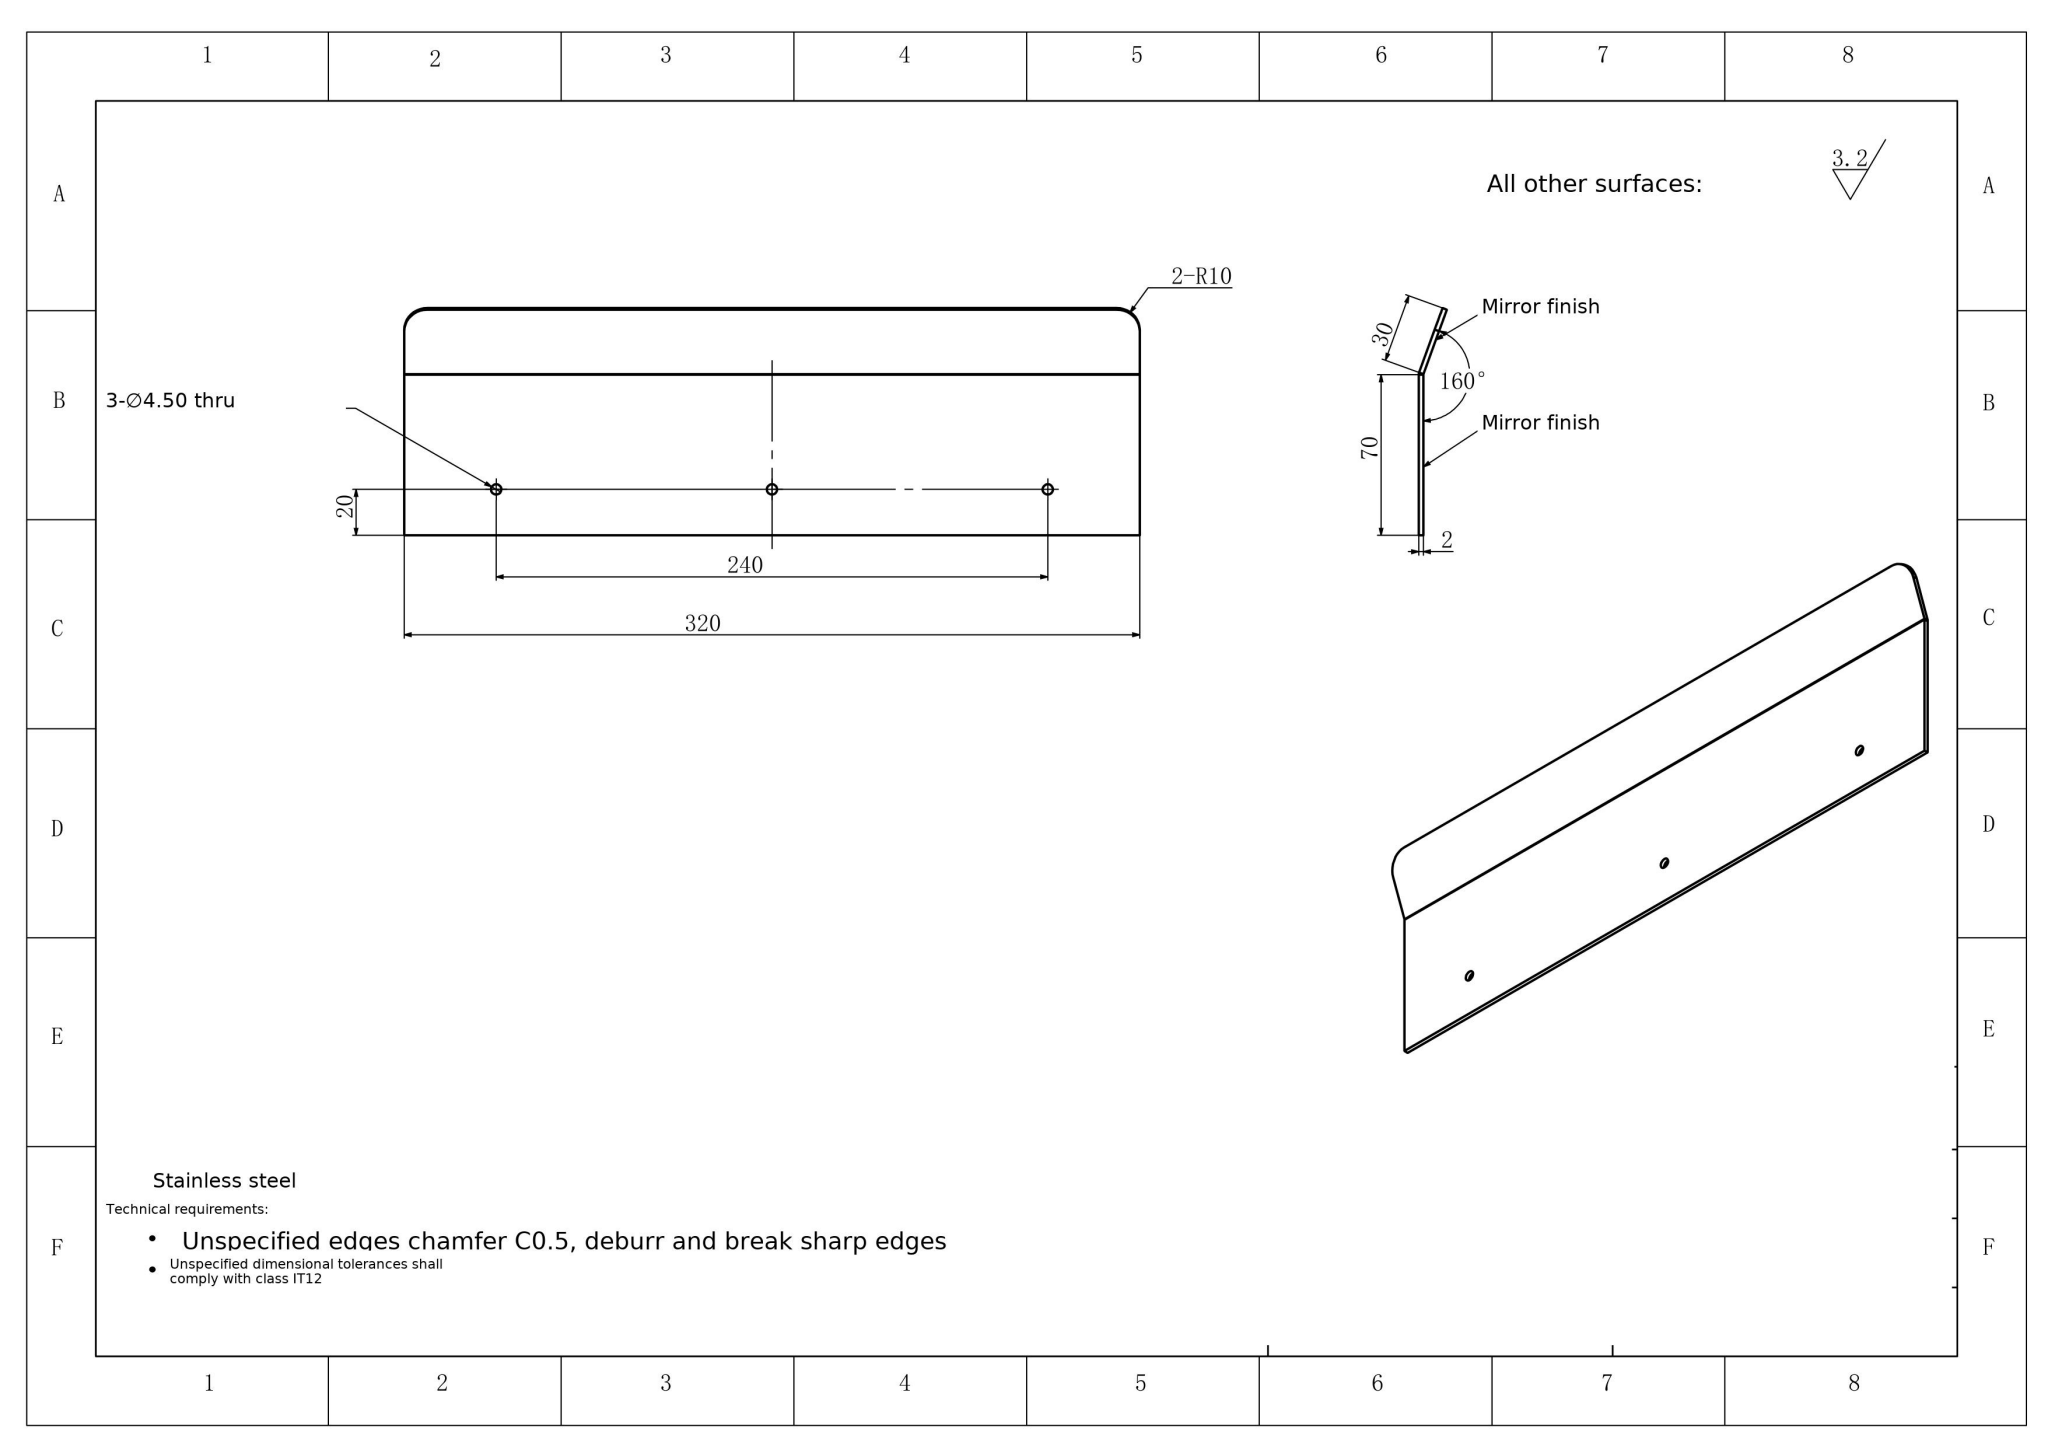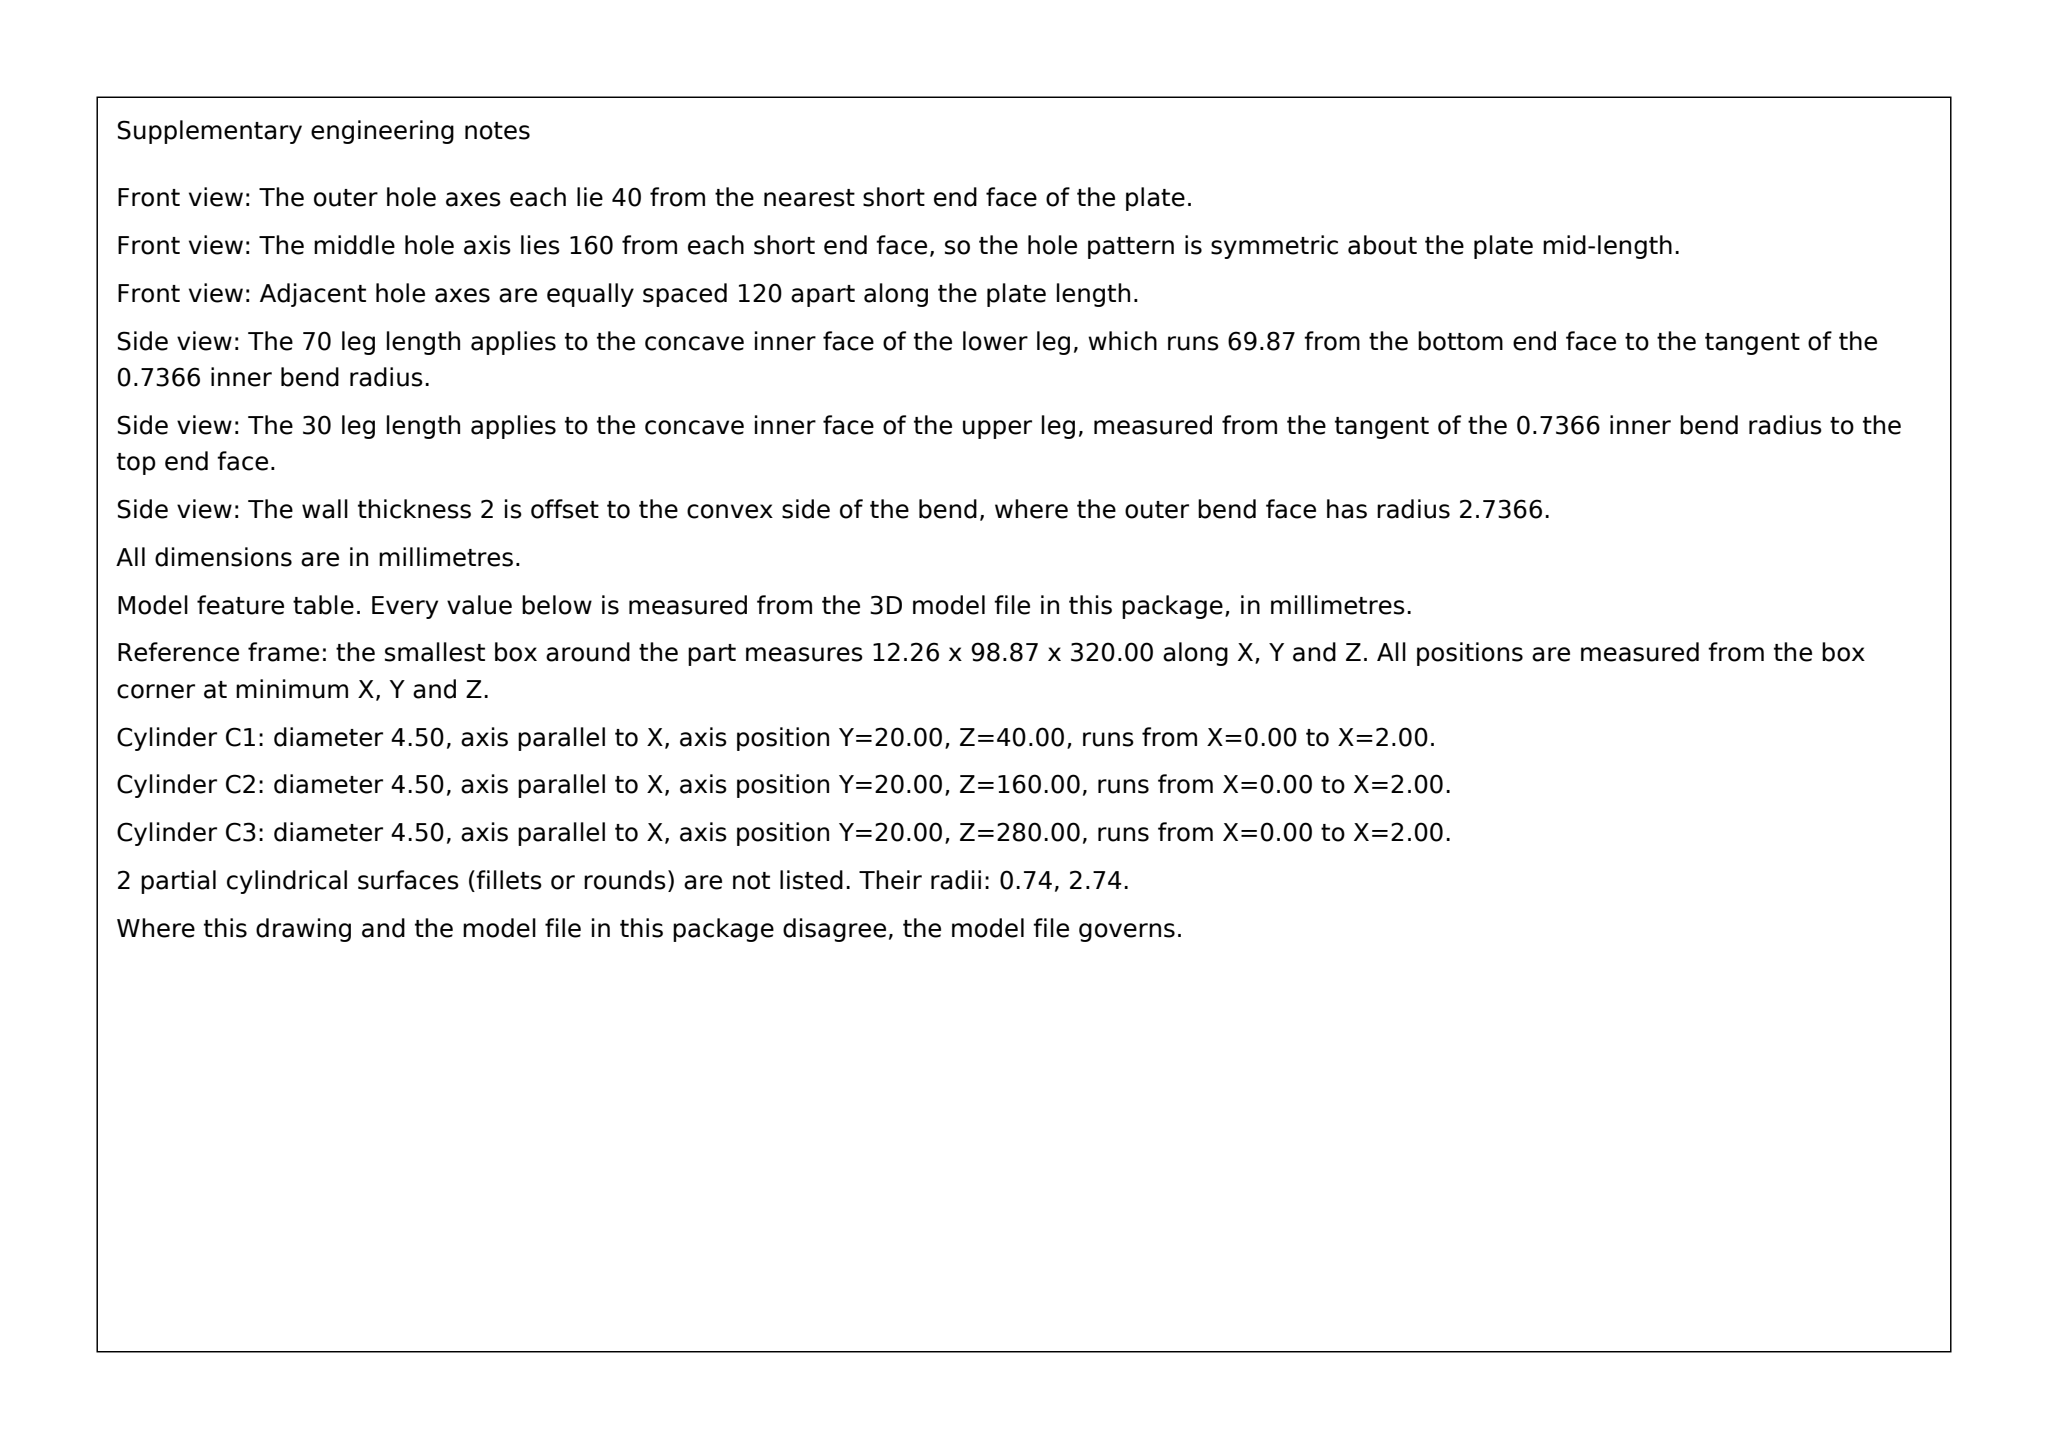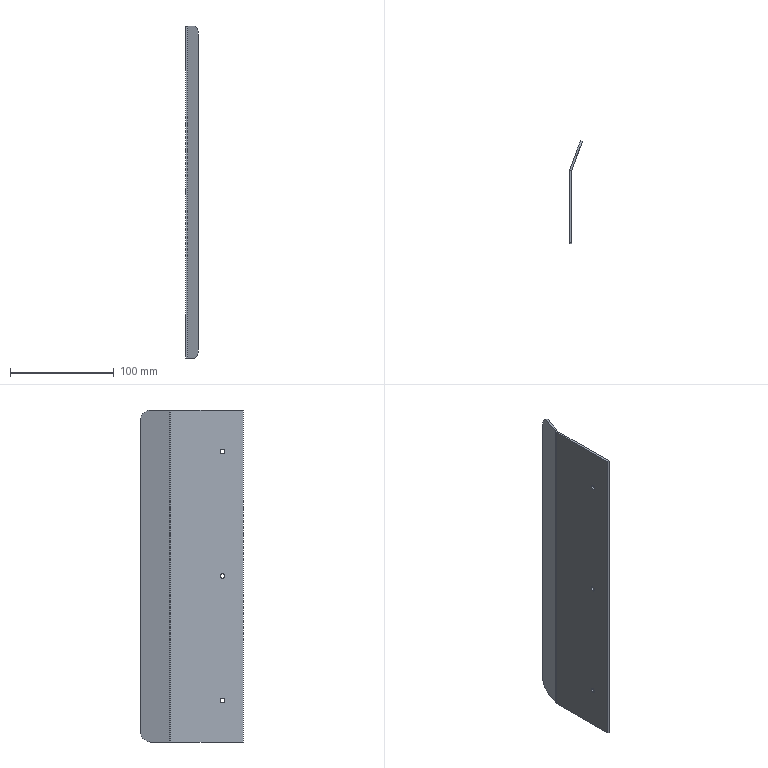Part | SolidWorks | mm | 1 solid | 22 faces | box 12.26 x 98.87 x 320 mm | volume 64040 mm3 | plane 12 | cylinder 10 | commonest cylinder face diameters 4.5 x6 20 x2 1.473 x1 5.473 x1
Drawing notes:
160° BEND: R0.74 INSIDE, R2.74 OUTSIDE | from the solid: cylinders dia 1.473 (r=0.7365) and 5.473 (r=2.736), axis z, len 320 at bend
ALL BENDS R0.74 INSIDE UNLESS NOTED; MATL THK 2 | from the solid: bend cyl dia 1.473 -> R0.74; planes x=0 and x=2.0 give 2 thk
STEP:
#1=CARTESIAN_POINT('',(-2.,-52.25,0.));
#2=VERTEX_POINT('',#1);
#3=CARTESIAN_POINT('',(-2.,-47.75,0.));
#4=VERTEX_POINT('',#3);
#5=CARTESIAN_POINT('',(-2.,-50.,0.));
#6=DIRECTION('',(1.,0.,0.));
#7=DIRECTION('',(-0.,1.,0.));
#8=AXIS2_PLACEMENT_3D('',#5,#6,#7);
#9=CIRCLE('',#8,2.25);
#10=EDGE_CURVE('',#2,#4,#9,.T.);
#11=ORIENTED_EDGE('',*,*,#10,.F.);
#12=CARTESIAN_POINT('',(0.,-52.25,0.));
#13=VERTEX_POINT('',#12);
#14=CARTESIAN_POINT('',(-10.,-52.25,0.));
#15=DIRECTION('',(1.,0.,0.));
#16=VECTOR('',#15,1000.);
#17=LINE('',#14,#16);
#18=EDGE_CURVE('',#2,#13,#17,.T.);
#19=ORIENTED_EDGE('',*,*,#18,.T.);
#20=CARTESIAN_POINT('',(0.,-47.75,0.));
#21=VERTEX_POINT('',#20);
#22=CARTESIAN_POINT('',(0.,-50.,0.));
#23=DIRECTION('',(1.,0.,0.));
#24=DIRECTION('',(-0.,1.,0.));
#25=AXIS2_PLACEMENT_3D('',#22,#23,#24);
#26=CIRCLE('',#25,2.25);
#27=EDGE_CURVE('',#13,#21,#26,.T.);
#28=ORIENTED_EDGE('',*,*,#27,.T.);
#29=CARTESIAN_POINT('',(-10.,-47.75,0.));
#30=DIRECTION('',(1.,0.,0.));
#31=VECTOR('',#30,1000.);
#32=LINE('',#29,#31);
#33=EDGE_CURVE('',#4,#21,#32,.T.);
#34=ORIENTED_EDGE('',*,*,#33,.F.);
#35=EDGE_LOOP('',(#11,#19,#28,#34));
#36=FACE_OUTER_BOUND('',#35,.T.);
#37=CARTESIAN_POINT('',(-10.,-50.,0.));
#38=DIRECTION('',(1.,0.,0.));
#39=DIRECTION('',(0.,1.,0.));
#40=AXIS2_PLACEMENT_3D('',#37,#38,#39);
#41=CYLINDRICAL_SURFACE('',#40,2.25);
#42=ADVANCED_FACE('',(#36),#41,.F.);
#43=CARTESIAN_POINT('',(-2.,-52.25,-120.));
#44=VERTEX_POINT('',#43);
#45=CARTESIAN_POINT('',(-2.,-47.75,-120.));
#46=VERTEX_POINT('',#45);
#47=CARTESIAN_POINT('',(-2.,-50.,-120.));
#48=DIRECTION('',(1.,0.,0.));
#49=DIRECTION('',(-0.,1.,0.));
#50=AXIS2_PLACEMENT_3D('',#47,#48,#49);
#51=CIRCLE('',#50,2.25);
#52=EDGE_CURVE('',#44,#46,#51,.T.);
#53=ORIENTED_EDGE('',*,*,#52,.F.);
#54=CARTESIAN_POINT('',(0.,-52.25,-120.));
#55=VERTEX_POINT('',#54);
#56=CARTESIAN_POINT('',(-10.,-52.25,-120.));
#57=DIRECTION('',(1.,0.,0.));
#58=VECTOR('',#57,1000.);
#59=LINE('',#56,#58);
#60=EDGE_CURVE('',#44,#55,#59,.T.);
#61=ORIENTED_EDGE('',*,*,#60,.T.);
#62=CARTESIAN_POINT('',(0.,-47.75,-120.));
#63=VERTEX_POINT('',#62);
#64=CARTESIAN_POINT('',(0.,-50.,-120.));
#65=DIRECTION('',(1.,0.,0.));
#66=DIRECTION('',(-0.,1.,0.));
#67=AXIS2_PLACEMENT_3D('',#64,#65,#66);
#68=CIRCLE('',#67,2.25);
#69=EDGE_CURVE('',#55,#63,#68,.T.);
#70=ORIENTED_EDGE('',*,*,#69,.T.);
#71=CARTESIAN_POINT('',(-10.,-47.75,-120.));
#72=DIRECTION('',(1.,0.,0.));
#73=VECTOR('',#72,1000.);
#74=LINE('',#71,#73);
#75=EDGE_CURVE('',#46,#63,#74,.T.);
#76=ORIENTED_EDGE('',*,*,#75,.F.);
#77=EDGE_LOOP('',(#53,#61,#70,#76));
#78=FACE_OUTER_BOUND('',#77,.T.);
#79=CARTESIAN_POINT('',(-10.,-50.,-120.));
#80=DIRECTION('',(1.,0.,0.));
#81=DIRECTION('',(0.,1.,0.));
#82=AXIS2_PLACEMENT_3D('',#79,#80,#81);
#83=CYLINDRICAL_SURFACE('',#82,2.25);
#84=ADVANCED_FACE('',(#78),#83,.F.);
#85=CARTESIAN_POINT('',(-2.,-52.25,120.));
#86=VERTEX_POINT('',#85);
#87=CARTESIAN_POINT('',(-2.,-47.75,120.));
#88=VERTEX_POINT('',#87);
#89=CARTESIAN_POINT('',(-2.,-50.,120.));
#90=DIRECTION('',(1.,0.,0.));
#91=DIRECTION('',(-0.,1.,0.));
#92=AXIS2_PLACEMENT_3D('',#89,#90,#91);
#93=CIRCLE('',#92,2.25);
#94=EDGE_CURVE('',#86,#88,#93,.T.);
#95=ORIENTED_EDGE('',*,*,#94,.F.);
#96=CARTESIAN_POINT('',(0.,-52.25,120.));
#97=VERTEX_POINT('',#96);
#98=CARTESIAN_POINT('',(-10.,-52.25,120.));
#99=DIRECTION('',(1.,0.,0.));
#100=VECTOR('',#99,1000.);
#101=LINE('',#98,#100);
#102=EDGE_CURVE('',#86,#97,#101,.T.);
#103=ORIENTED_EDGE('',*,*,#102,.T.);
#104=CARTESIAN_POINT('',(0.,-47.75,120.));
#105=VERTEX_POINT('',#104);
#106=CARTESIAN_POINT('',(0.,-50.,120.));
#107=DIRECTION('',(1.,0.,0.));
#108=DIRECTION('',(-0.,1.,0.));
#109=AXIS2_PLACEMENT_3D('',#106,#107,#108);
#110=CIRCLE('',#109,2.25);
#111=EDGE_CURVE('',#97,#105,#110,.T.);
#112=ORIENTED_EDGE('',*,*,#111,.T.);
#113=CARTESIAN_POINT('',(-10.,-47.75,120.));
#114=DIRECTION('',(1.,0.,0.));
#115=VECTOR('',#114,1000.);
#116=LINE('',#113,#115);
#117=EDGE_CURVE('',#88,#105,#116,.T.);
#118=ORIENTED_EDGE('',*,*,#117,.F.);
#119=EDGE_LOOP('',(#95,#103,#112,#118));
#120=FACE_OUTER_BOUND('',#119,.T.);
#121=CARTESIAN_POINT('',(-10.,-50.,120.));
#122=DIRECTION('',(1.,0.,0.));
#123=DIRECTION('',(0.,1.,0.));
#124=AXIS2_PLACEMENT_3D('',#121,#122,#123);
#125=CYLINDRICAL_SURFACE('',#124,2.25);
#126=ADVANCED_FACE('',(#120),#125,.F.);
#127=CARTESIAN_POINT('',(0.,-0.1299,160.));
#128=VERTEX_POINT('',#127);
#129=CARTESIAN_POINT('',(-2.,-0.1299,160.));
#130=VERTEX_POINT('',#129);
#131=CARTESIAN_POINT('',(0.,-0.1299,160.));
#132=DIRECTION('',(-1.,-0.,0.));
#133=VECTOR('',#132,1000.);
#134=LINE('',#131,#133);
#135=EDGE_CURVE('',#128,#130,#134,.T.);
#136=ORIENTED_EDGE('',*,*,#135,.F.);
#137=CARTESIAN_POINT('',(0.04442,0.122,160.));
#138=VERTEX_POINT('',#137);
#139=CARTESIAN_POINT('',(0.7366,-0.1299,160.));
#140=DIRECTION('',(0.,0.,1.));
#141=DIRECTION('',(-1.,0.,0.));
#142=AXIS2_PLACEMENT_3D('',#139,#140,#141);
#143=CIRCLE('',#142,0.7366);
#144=EDGE_CURVE('',#138,#128,#143,.T.);
#145=ORIENTED_EDGE('',*,*,#144,.F.);
#146=CARTESIAN_POINT('',(-1.835,0.8061,160.));
#147=VERTEX_POINT('',#146);
#148=CARTESIAN_POINT('',(-1.835,0.8061,160.));
#149=DIRECTION('',(0.9397,-0.342,0.));
#150=VECTOR('',#149,1000.);
#151=LINE('',#148,#150);
#152=EDGE_CURVE('',#147,#138,#151,.T.);
#153=ORIENTED_EDGE('',*,*,#152,.F.);
#154=CARTESIAN_POINT('',(0.7366,-0.1299,160.));
#155=DIRECTION('',(0.,0.,1.));
#156=DIRECTION('',(1.,0.,0.));
#157=AXIS2_PLACEMENT_3D('',#154,#155,#156);
#158=CIRCLE('',#157,2.737);
#159=EDGE_CURVE('',#147,#130,#158,.T.);
#160=ORIENTED_EDGE('',*,*,#159,.T.);
#161=EDGE_LOOP('',(#136,#145,#153,#160));
#162=FACE_OUTER_BOUND('',#161,.T.);
#163=CARTESIAN_POINT('',(0.,-0.1299,160.));
#164=DIRECTION('',(0.,0.,1.));
#165=DIRECTION('',(1.,0.,0.));
#166=AXIS2_PLACEMENT_3D('',#163,#164,#165);
#167=PLANE('',#166);
#168=ADVANCED_FACE('',(#162),#167,.T.);
#169=CARTESIAN_POINT('',(0.,-70.,160.));
#170=VERTEX_POINT('',#169);
#171=CARTESIAN_POINT('',(0.,0.,160.));
#172=DIRECTION('',(0.,-1.,0.));
#173=VECTOR('',#172,1000.);
#174=LINE('',#171,#173);
#175=EDGE_CURVE('',#128,#170,#174,.T.);
#176=ORIENTED_EDGE('',*,*,#175,.F.);
#177=ORIENTED_EDGE('',*,*,#135,.T.);
#178=CARTESIAN_POINT('',(-2.,-70.,160.));
#179=VERTEX_POINT('',#178);
#180=CARTESIAN_POINT('',(-2.,-0.,160.));
#181=DIRECTION('',(0.,-1.,0.));
#182=VECTOR('',#181,1000.);
#183=LINE('',#180,#182);
#184=EDGE_CURVE('',#130,#179,#183,.T.);
#185=ORIENTED_EDGE('',*,*,#184,.T.);
#186=CARTESIAN_POINT('',(0.,-70.,160.));
#187=DIRECTION('',(-1.,0.,0.));
#188=VECTOR('',#187,1000.);
#189=LINE('',#186,#188);
#190=EDGE_CURVE('',#170,#179,#189,.T.);
#191=ORIENTED_EDGE('',*,*,#190,.F.);
#192=EDGE_LOOP('',(#176,#177,#185,#191));
#193=FACE_OUTER_BOUND('',#192,.T.);
#194=CARTESIAN_POINT('',(-1.835,0.8061,160.));
#195=DIRECTION('',(0.,0.,1.));
#196=DIRECTION('',(1.,0.,0.));
#197=AXIS2_PLACEMENT_3D('',#194,#195,#196);
#198=PLANE('',#197);
#199=ADVANCED_FACE('',(#193),#198,.T.);
#200=CARTESIAN_POINT('',(0.04442,0.122,-160.));
#201=VERTEX_POINT('',#200);
#202=CARTESIAN_POINT('',(-1.835,0.8061,-160.));
#203=VERTEX_POINT('',#202);
#204=CARTESIAN_POINT('',(0.04442,0.122,-160.));
#205=DIRECTION('',(-0.9397,0.342,0.));
#206=VECTOR('',#205,1000.);
#207=LINE('',#204,#206);
#208=EDGE_CURVE('',#201,#203,#207,.T.);
#209=ORIENTED_EDGE('',*,*,#208,.F.);
#210=CARTESIAN_POINT('',(0.,-0.1299,-160.));
#211=VERTEX_POINT('',#210);
#212=CARTESIAN_POINT('',(0.7366,-0.1299,-160.));
#213=DIRECTION('',(0.,0.,1.));
#214=DIRECTION('',(-1.,0.,0.));
#215=AXIS2_PLACEMENT_3D('',#212,#213,#214);
#216=CIRCLE('',#215,0.7366);
#217=EDGE_CURVE('',#201,#211,#216,.T.);
#218=ORIENTED_EDGE('',*,*,#217,.T.);
#219=CARTESIAN_POINT('',(-2.,-0.1299,-160.));
#220=VERTEX_POINT('',#219);
#221=CARTESIAN_POINT('',(-2.,-0.1299,-160.));
#222=DIRECTION('',(1.,0.,0.));
#223=VECTOR('',#222,1000.);
#224=LINE('',#221,#223);
#225=EDGE_CURVE('',#220,#211,#224,.T.);
#226=ORIENTED_EDGE('',*,*,#225,.F.);
#227=CARTESIAN_POINT('',(0.7366,-0.1299,-160.));
#228=DIRECTION('',(0.,0.,1.));
#229=DIRECTION('',(1.,0.,0.));
#230=AXIS2_PLACEMENT_3D('',#227,#228,#229);
#231=CIRCLE('',#230,2.737);
#232=EDGE_CURVE('',#203,#220,#231,.T.);
#233=ORIENTED_EDGE('',*,*,#232,.F.);
#234=EDGE_LOOP('',(#209,#218,#226,#233));
#235=FACE_OUTER_BOUND('',#234,.T.);
#236=CARTESIAN_POINT('',(0.04442,0.122,-160.));
#237=DIRECTION('',(0.,0.,-1.));
#238=DIRECTION('',(-1.,0.,0.));
#239=AXIS2_PLACEMENT_3D('',#236,#237,#238);
#240=PLANE('',#239);
#241=ADVANCED_FACE('',(#235),#240,.T.);
#242=CARTESIAN_POINT('',(4.961,19.478,-160.));
#243=VERTEX_POINT('',#242);
#244=CARTESIAN_POINT('',(-1.879,0.684,-160.));
#245=DIRECTION('',(-0.342,-0.9397,0.));
#246=VECTOR('',#245,1000.);
#247=LINE('',#244,#246);
#248=EDGE_CURVE('',#243,#203,#247,.T.);
#249=ORIENTED_EDGE('',*,*,#248,.F.);
#250=CARTESIAN_POINT('',(6.84,18.794,-160.));
#251=VERTEX_POINT('',#250);
#252=CARTESIAN_POINT('',(5.116,19.421,-160.));
#253=DIRECTION('',(0.9397,-0.342,0.));
#254=VECTOR('',#253,1000.);
#255=LINE('',#252,#254);
#256=EDGE_CURVE('',#243,#251,#255,.T.);
#257=ORIENTED_EDGE('',*,*,#256,.T.);
#258=CARTESIAN_POINT('',(0.,0.,-160.));
#259=DIRECTION('',(-0.342,-0.9397,0.));
#260=VECTOR('',#259,1000.);
#261=LINE('',#258,#260);
#262=EDGE_CURVE('',#251,#201,#261,.T.);
#263=ORIENTED_EDGE('',*,*,#262,.T.);
#264=ORIENTED_EDGE('',*,*,#208,.T.);
#265=EDGE_LOOP('',(#249,#257,#263,#264));
#266=FACE_OUTER_BOUND('',#265,.T.);
#267=CARTESIAN_POINT('',(-2.,-0.1299,-160.));
#268=DIRECTION('',(0.,0.,-1.));
#269=DIRECTION('',(-1.,0.,0.));
#270=AXIS2_PLACEMENT_3D('',#267,#268,#269);
#271=PLANE('',#270);
#272=ADVANCED_FACE('',(#266),#271,.T.);
#273=CARTESIAN_POINT('',(-2.,-50.,0.));
#274=DIRECTION('',(1.,0.,0.));
#275=DIRECTION('',(-0.,1.,0.));
#276=AXIS2_PLACEMENT_3D('',#273,#274,#275);
#277=CIRCLE('',#276,2.25);
#278=EDGE_CURVE('',#4,#2,#277,.T.);
#279=ORIENTED_EDGE('',*,*,#278,.T.);
#280=ORIENTED_EDGE('',*,*,#10,.T.);
#281=EDGE_LOOP('',(#279,#280));
#282=FACE_BOUND('',#281,.T.);
#283=CARTESIAN_POINT('',(-2.,-50.,-120.));
#284=DIRECTION('',(1.,0.,0.));
#285=DIRECTION('',(-0.,1.,0.));
#286=AXIS2_PLACEMENT_3D('',#283,#284,#285);
#287=CIRCLE('',#286,2.25);
#288=EDGE_CURVE('',#46,#44,#287,.T.);
#289=ORIENTED_EDGE('',*,*,#288,.T.);
#290=ORIENTED_EDGE('',*,*,#52,.T.);
#291=EDGE_LOOP('',(#289,#290));
#292=FACE_BOUND('',#291,.T.);
#293=CARTESIAN_POINT('',(-2.,-50.,120.));
#294=DIRECTION('',(1.,0.,0.));
#295=DIRECTION('',(-0.,1.,0.));
#296=AXIS2_PLACEMENT_3D('',#293,#294,#295);
#297=CIRCLE('',#296,2.25);
#298=EDGE_CURVE('',#88,#86,#297,.T.);
#299=ORIENTED_EDGE('',*,*,#298,.T.);
#300=ORIENTED_EDGE('',*,*,#94,.T.);
#301=EDGE_LOOP('',(#299,#300));
#302=FACE_BOUND('',#301,.T.);
#303=CARTESIAN_POINT('',(-2.,-70.,-160.));
#304=VERTEX_POINT('',#303);
#305=CARTESIAN_POINT('',(-2.,-0.,-160.));
#306=DIRECTION('',(0.,-1.,0.));
#307=VECTOR('',#306,1000.);
#308=LINE('',#305,#307);
#309=EDGE_CURVE('',#220,#304,#308,.T.);
#310=ORIENTED_EDGE('',*,*,#309,.T.);
#311=CARTESIAN_POINT('',(-2.,-70.,160.));
#312=DIRECTION('',(0.,0.,-1.));
#313=VECTOR('',#312,1000.);
#314=LINE('',#311,#313);
#315=EDGE_CURVE('',#179,#304,#314,.T.);
#316=ORIENTED_EDGE('',*,*,#315,.F.);
#317=ORIENTED_EDGE('',*,*,#184,.F.);
#318=CARTESIAN_POINT('',(-2.,-0.1299,160.));
#319=DIRECTION('',(0.,0.,-1.));
#320=VECTOR('',#319,1000.);
#321=LINE('',#318,#320);
#322=EDGE_CURVE('',#130,#220,#321,.T.);
#323=ORIENTED_EDGE('',*,*,#322,.T.);
#324=EDGE_LOOP('',(#310,#316,#317,#323));
#325=FACE_OUTER_BOUND('',#324,.T.);
#326=CARTESIAN_POINT('',(-2.,-0.,160.));
#327=DIRECTION('',(1.,0.,0.));
#328=DIRECTION('',(-0.,1.,0.));
#329=AXIS2_PLACEMENT_3D('',#326,#327,#328);
#330=PLANE('',#329);
#331=ADVANCED_FACE('',(#282,#292,#302,#325),#330,.F.);
#332=CARTESIAN_POINT('',(0.,-70.,-160.));
#333=VERTEX_POINT('',#332);
#334=CARTESIAN_POINT('',(0.,-70.,-160.));
#335=DIRECTION('',(-1.,0.,0.));
#336=VECTOR('',#335,1000.);
#337=LINE('',#334,#336);
#338=EDGE_CURVE('',#333,#304,#337,.T.);
#339=ORIENTED_EDGE('',*,*,#338,.F.);
#340=CARTESIAN_POINT('',(0.,-70.,160.));
#341=DIRECTION('',(0.,0.,-1.));
#342=VECTOR('',#341,1000.);
#343=LINE('',#340,#342);
#344=EDGE_CURVE('',#170,#333,#343,.T.);
#345=ORIENTED_EDGE('',*,*,#344,.F.);
#346=ORIENTED_EDGE('',*,*,#190,.T.);
#347=ORIENTED_EDGE('',*,*,#315,.T.);
#348=EDGE_LOOP('',(#339,#345,#346,#347));
#349=FACE_OUTER_BOUND('',#348,.T.);
#350=CARTESIAN_POINT('',(0.,-70.,160.));
#351=DIRECTION('',(0.,-1.,0.));
#352=DIRECTION('',(0.,0.,-1.));
#353=AXIS2_PLACEMENT_3D('',#350,#351,#352);
#354=PLANE('',#353);
#355=ADVANCED_FACE('',(#349),#354,.T.);
#356=CARTESIAN_POINT('',(0.,-50.,0.));
#357=DIRECTION('',(1.,0.,0.));
#358=DIRECTION('',(-0.,1.,0.));
#359=AXIS2_PLACEMENT_3D('',#356,#357,#358);
#360=CIRCLE('',#359,2.25);
#361=EDGE_CURVE('',#21,#13,#360,.T.);
#362=ORIENTED_EDGE('',*,*,#361,.F.);
#363=ORIENTED_EDGE('',*,*,#27,.F.);
#364=EDGE_LOOP('',(#362,#363));
#365=FACE_BOUND('',#364,.T.);
#366=CARTESIAN_POINT('',(0.,-50.,-120.));
#367=DIRECTION('',(1.,0.,0.));
#368=DIRECTION('',(-0.,1.,0.));
#369=AXIS2_PLACEMENT_3D('',#366,#367,#368);
#370=CIRCLE('',#369,2.25);
#371=EDGE_CURVE('',#63,#55,#370,.T.);
#372=ORIENTED_EDGE('',*,*,#371,.F.);
#373=ORIENTED_EDGE('',*,*,#69,.F.);
#374=EDGE_LOOP('',(#372,#373));
#375=FACE_BOUND('',#374,.T.);
#376=CARTESIAN_POINT('',(0.,-50.,120.));
#377=DIRECTION('',(1.,0.,0.));
#378=DIRECTION('',(-0.,1.,0.));
#379=AXIS2_PLACEMENT_3D('',#376,#377,#378);
#380=CIRCLE('',#379,2.25);
#381=EDGE_CURVE('',#105,#97,#380,.T.);
#382=ORIENTED_EDGE('',*,*,#381,.F.);
#383=ORIENTED_EDGE('',*,*,#111,.F.);
#384=EDGE_LOOP('',(#382,#383));
#385=FACE_BOUND('',#384,.T.);
#386=CARTESIAN_POINT('',(0.,0.,-160.));
#387=DIRECTION('',(0.,-1.,0.));
#388=VECTOR('',#387,1000.);
#389=LINE('',#386,#388);
#390=EDGE_CURVE('',#211,#333,#389,.T.);
#391=ORIENTED_EDGE('',*,*,#390,.F.);
#392=CARTESIAN_POINT('',(0.,-0.1299,160.));
#393=DIRECTION('',(0.,0.,-1.));
#394=VECTOR('',#393,1000.);
#395=LINE('',#392,#394);
#396=EDGE_CURVE('',#128,#211,#395,.T.);
#397=ORIENTED_EDGE('',*,*,#396,.F.);
#398=ORIENTED_EDGE('',*,*,#175,.T.);
#399=ORIENTED_EDGE('',*,*,#344,.T.);
#400=EDGE_LOOP('',(#391,#397,#398,#399));
#401=FACE_OUTER_BOUND('',#400,.T.);
#402=CARTESIAN_POINT('',(0.,0.,160.));
#403=DIRECTION('',(1.,0.,0.));
#404=DIRECTION('',(-0.,1.,0.));
#405=AXIS2_PLACEMENT_3D('',#402,#403,#404);
#406=PLANE('',#405);
#407=ADVANCED_FACE('',(#365,#375,#385,#401),#406,.T.);
#408=ORIENTED_EDGE('',*,*,#217,.F.);
#409=CARTESIAN_POINT('',(0.04442,0.122,160.));
#410=DIRECTION('',(0.,0.,-1.));
#411=VECTOR('',#410,1000.);
#412=LINE('',#409,#411);
#413=EDGE_CURVE('',#138,#201,#412,.T.);
#414=ORIENTED_EDGE('',*,*,#413,.F.);
#415=ORIENTED_EDGE('',*,*,#144,.T.);
#416=ORIENTED_EDGE('',*,*,#396,.T.);
#417=EDGE_LOOP('',(#408,#414,#415,#416));
#418=FACE_OUTER_BOUND('',#417,.T.);
#419=CARTESIAN_POINT('',(0.7366,-0.1299,160.));
#420=DIRECTION('',(0.,0.,-1.));
#421=DIRECTION('',(-1.,0.,0.));
#422=AXIS2_PLACEMENT_3D('',#419,#420,#421);
#423=CYLINDRICAL_SURFACE('',#422,0.7366);
#424=ADVANCED_FACE('',(#418),#423,.F.);
#425=ORIENTED_EDGE('',*,*,#262,.F.);
#426=CARTESIAN_POINT('',(10.261,28.191,-150.));
#427=VERTEX_POINT('',#426);
#428=CARTESIAN_POINT('',(6.84,18.794,-150.));
#429=DIRECTION('',(0.9397,-0.342,0.));
#430=DIRECTION('',(0.342,0.9397,0.));
#431=AXIS2_PLACEMENT_3D('',#428,#429,#430);
#432=CIRCLE('',#431,10.);
#433=EDGE_CURVE('',#251,#427,#432,.T.);
#434=ORIENTED_EDGE('',*,*,#433,.T.);
#435=CARTESIAN_POINT('',(10.261,28.191,150.));
#436=VERTEX_POINT('',#435);
#437=CARTESIAN_POINT('',(10.261,28.191,160.));
#438=DIRECTION('',(0.,0.,-1.));
#439=VECTOR('',#438,1000.);
#440=LINE('',#437,#439);
#441=EDGE_CURVE('',#436,#427,#440,.T.);
#442=ORIENTED_EDGE('',*,*,#441,.F.);
#443=CARTESIAN_POINT('',(6.84,18.794,160.));
#444=VERTEX_POINT('',#443);
#445=CARTESIAN_POINT('',(6.84,18.794,150.));
#446=DIRECTION('',(0.9397,-0.342,0.));
#447=DIRECTION('',(0.342,0.9397,0.));
#448=AXIS2_PLACEMENT_3D('',#445,#446,#447);
#449=CIRCLE('',#448,10.);
#450=EDGE_CURVE('',#436,#444,#449,.T.);
#451=ORIENTED_EDGE('',*,*,#450,.T.);
#452=CARTESIAN_POINT('',(0.,0.,160.));
#453=DIRECTION('',(-0.342,-0.9397,0.));
#454=VECTOR('',#453,1000.);
#455=LINE('',#452,#454);
#456=EDGE_CURVE('',#444,#138,#455,.T.);
#457=ORIENTED_EDGE('',*,*,#456,.T.);
#458=ORIENTED_EDGE('',*,*,#413,.T.);
#459=EDGE_LOOP('',(#425,#434,#442,#451,#457,#458));
#460=FACE_OUTER_BOUND('',#459,.T.);
#461=CARTESIAN_POINT('',(0.,0.,160.));
#462=DIRECTION('',(0.9397,-0.342,0.));
#463=DIRECTION('',(0.342,0.9397,0.));
#464=AXIS2_PLACEMENT_3D('',#461,#462,#463);
#465=PLANE('',#464);
#466=ADVANCED_FACE('',(#460),#465,.T.);
#467=ORIENTED_EDGE('',*,*,#441,.T.);
#468=CARTESIAN_POINT('',(8.381,28.875,-150.));
#469=VERTEX_POINT('',#468);
#470=CARTESIAN_POINT('',(8.381,28.875,-150.));
#471=DIRECTION('',(-0.9397,0.342,0.));
#472=VECTOR('',#471,1000.);
#473=LINE('',#470,#472);
#474=EDGE_CURVE('',#427,#469,#473,.T.);
#475=ORIENTED_EDGE('',*,*,#474,.T.);
#476=CARTESIAN_POINT('',(8.381,28.875,150.));
#477=VERTEX_POINT('',#476);
#478=CARTESIAN_POINT('',(8.381,28.875,160.));
#479=DIRECTION('',(0.,0.,-1.));
#480=VECTOR('',#479,1000.);
#481=LINE('',#478,#480);
#482=EDGE_CURVE('',#477,#469,#481,.T.);
#483=ORIENTED_EDGE('',*,*,#482,.F.);
#484=CARTESIAN_POINT('',(10.261,28.191,150.));
#485=DIRECTION('',(0.9397,-0.342,0.));
#486=VECTOR('',#485,1000.);
#487=LINE('',#484,#486);
#488=EDGE_CURVE('',#477,#436,#487,.T.);
#489=ORIENTED_EDGE('',*,*,#488,.T.);
#490=EDGE_LOOP('',(#467,#475,#483,#489));
#491=FACE_OUTER_BOUND('',#490,.T.);
#492=CARTESIAN_POINT('',(8.381,28.875,160.));
#493=DIRECTION('',(0.342,0.9397,0.));
#494=DIRECTION('',(-0.9397,0.342,0.));
#495=AXIS2_PLACEMENT_3D('',#492,#493,#494);
#496=PLANE('',#495);
#497=ADVANCED_FACE('',(#491),#496,.T.);
#498=ORIENTED_EDGE('',*,*,#482,.T.);
#499=CARTESIAN_POINT('',(4.961,19.478,-150.));
#500=DIRECTION('',(-0.9397,0.342,0.));
#501=DIRECTION('',(0.342,0.9397,0.));
#502=AXIS2_PLACEMENT_3D('',#499,#500,#501);
#503=CIRCLE('',#502,10.);
#504=EDGE_CURVE('',#469,#243,#503,.T.);
#505=ORIENTED_EDGE('',*,*,#504,.T.);
#506=ORIENTED_EDGE('',*,*,#248,.T.);
#507=CARTESIAN_POINT('',(-1.835,0.8061,160.));
#508=DIRECTION('',(0.,0.,-1.));
#509=VECTOR('',#508,1000.);
#510=LINE('',#507,#509);
#511=EDGE_CURVE('',#147,#203,#510,.T.);
#512=ORIENTED_EDGE('',*,*,#511,.F.);
#513=CARTESIAN_POINT('',(4.961,19.478,160.));
#514=VERTEX_POINT('',#513);
#515=CARTESIAN_POINT('',(-1.879,0.684,160.));
#516=DIRECTION('',(-0.342,-0.9397,0.));
#517=VECTOR('',#516,1000.);
#518=LINE('',#515,#517);
#519=EDGE_CURVE('',#514,#147,#518,.T.);
#520=ORIENTED_EDGE('',*,*,#519,.F.);
#521=CARTESIAN_POINT('',(4.961,19.478,150.));
#522=DIRECTION('',(-0.9397,0.342,0.));
#523=DIRECTION('',(0.342,0.9397,0.));
#524=AXIS2_PLACEMENT_3D('',#521,#522,#523);
#525=CIRCLE('',#524,10.);
#526=EDGE_CURVE('',#514,#477,#525,.T.);
#527=ORIENTED_EDGE('',*,*,#526,.T.);
#528=EDGE_LOOP('',(#498,#505,#506,#512,#520,#527));
#529=FACE_OUTER_BOUND('',#528,.T.);
#530=CARTESIAN_POINT('',(-1.879,0.684,160.));
#531=DIRECTION('',(0.9397,-0.342,0.));
#532=DIRECTION('',(0.342,0.9397,0.));
#533=AXIS2_PLACEMENT_3D('',#530,#531,#532);
#534=PLANE('',#533);
#535=ADVANCED_FACE('',(#529),#534,.F.);
#536=ORIENTED_EDGE('',*,*,#232,.T.);
#537=ORIENTED_EDGE('',*,*,#322,.F.);
#538=ORIENTED_EDGE('',*,*,#159,.F.);
#539=ORIENTED_EDGE('',*,*,#511,.T.);
#540=EDGE_LOOP('',(#536,#537,#538,#539));
#541=FACE_OUTER_BOUND('',#540,.T.);
#542=CARTESIAN_POINT('',(0.7366,-0.1299,160.));
#543=DIRECTION('',(0.,0.,-1.));
#544=DIRECTION('',(-1.,0.,0.));
#545=AXIS2_PLACEMENT_3D('',#542,#543,#544);
#546=CYLINDRICAL_SURFACE('',#545,2.737);
#547=ADVANCED_FACE('',(#541),#546,.T.);
#548=ORIENTED_EDGE('',*,*,#456,.F.);
#549=CARTESIAN_POINT('',(4.961,19.478,160.));
#550=DIRECTION('',(-0.9397,0.342,0.));
#551=VECTOR('',#550,1000.);
#552=LINE('',#549,#551);
#553=EDGE_CURVE('',#444,#514,#552,.T.);
#554=ORIENTED_EDGE('',*,*,#553,.T.);
#555=ORIENTED_EDGE('',*,*,#519,.T.);
#556=ORIENTED_EDGE('',*,*,#152,.T.);
#557=EDGE_LOOP('',(#548,#554,#555,#556));
#558=FACE_OUTER_BOUND('',#557,.T.);
#559=CARTESIAN_POINT('',(0.7366,-0.1299,160.));
#560=DIRECTION('',(0.,0.,-1.));
#561=DIRECTION('',(-1.,0.,0.));
#562=AXIS2_PLACEMENT_3D('',#559,#560,#561);
#563=PLANE('',#562);
#564=ADVANCED_FACE('',(#558),#563,.F.);
#565=ORIENTED_EDGE('',*,*,#309,.F.);
#566=ORIENTED_EDGE('',*,*,#225,.T.);
#567=ORIENTED_EDGE('',*,*,#390,.T.);
#568=ORIENTED_EDGE('',*,*,#338,.T.);
#569=EDGE_LOOP('',(#565,#566,#567,#568));
#570=FACE_OUTER_BOUND('',#569,.T.);
#571=CARTESIAN_POINT('',(0.7366,-0.1299,-160.));
#572=DIRECTION('',(0.,0.,-1.));
#573=DIRECTION('',(-1.,0.,0.));
#574=AXIS2_PLACEMENT_3D('',#571,#572,#573);
#575=PLANE('',#574);
#576=ADVANCED_FACE('',(#570),#575,.T.);
#577=ORIENTED_EDGE('',*,*,#102,.F.);
#578=ORIENTED_EDGE('',*,*,#298,.F.);
#579=ORIENTED_EDGE('',*,*,#117,.T.);
#580=ORIENTED_EDGE('',*,*,#381,.T.);
#581=EDGE_LOOP('',(#577,#578,#579,#580));
#582=FACE_OUTER_BOUND('',#581,.T.);
#583=CARTESIAN_POINT('',(-10.,-50.,120.));
#584=DIRECTION('',(1.,0.,0.));
#585=DIRECTION('',(0.,1.,0.));
#586=AXIS2_PLACEMENT_3D('',#583,#584,#585);
#587=CYLINDRICAL_SURFACE('',#586,2.25);
#588=ADVANCED_FACE('',(#582),#587,.F.);
#589=ORIENTED_EDGE('',*,*,#60,.F.);
#590=ORIENTED_EDGE('',*,*,#288,.F.);
#591=ORIENTED_EDGE('',*,*,#75,.T.);
#592=ORIENTED_EDGE('',*,*,#371,.T.);
#593=EDGE_LOOP('',(#589,#590,#591,#592));
#594=FACE_OUTER_BOUND('',#593,.T.);
#595=CARTESIAN_POINT('',(-10.,-50.,-120.));
#596=DIRECTION('',(1.,0.,0.));
#597=DIRECTION('',(0.,1.,0.));
#598=AXIS2_PLACEMENT_3D('',#595,#596,#597);
#599=CYLINDRICAL_SURFACE('',#598,2.25);
#600=ADVANCED_FACE('',(#594),#599,.F.);
#601=ORIENTED_EDGE('',*,*,#18,.F.);
#602=ORIENTED_EDGE('',*,*,#278,.F.);
#603=ORIENTED_EDGE('',*,*,#33,.T.);
#604=ORIENTED_EDGE('',*,*,#361,.T.);
#605=EDGE_LOOP('',(#601,#602,#603,#604));
#606=FACE_OUTER_BOUND('',#605,.T.);
#607=CARTESIAN_POINT('',(-10.,-50.,0.));
#608=DIRECTION('',(1.,0.,0.));
#609=DIRECTION('',(0.,1.,0.));
#610=AXIS2_PLACEMENT_3D('',#607,#608,#609);
#611=CYLINDRICAL_SURFACE('',#610,2.25);
#612=ADVANCED_FACE('',(#606),#611,.F.);
#613=ORIENTED_EDGE('',*,*,#504,.F.);
#614=ORIENTED_EDGE('',*,*,#474,.F.);
#615=ORIENTED_EDGE('',*,*,#433,.F.);
#616=ORIENTED_EDGE('',*,*,#256,.F.);
#617=EDGE_LOOP('',(#613,#614,#615,#616));
#618=FACE_OUTER_BOUND('',#617,.T.);
#619=CARTESIAN_POINT('',(5.116,19.421,-150.));
#620=DIRECTION('',(0.9397,-0.342,0.));
#621=DIRECTION('',(0.342,0.9397,0.));
#622=AXIS2_PLACEMENT_3D('',#619,#620,#621);
#623=CYLINDRICAL_SURFACE('',#622,10.);
#624=ADVANCED_FACE('',(#618),#623,.T.);
#625=ORIENTED_EDGE('',*,*,#526,.F.);
#626=ORIENTED_EDGE('',*,*,#553,.F.);
#627=ORIENTED_EDGE('',*,*,#450,.F.);
#628=ORIENTED_EDGE('',*,*,#488,.F.);
#629=EDGE_LOOP('',(#625,#626,#627,#628));
#630=FACE_OUTER_BOUND('',#629,.T.);
#631=CARTESIAN_POINT('',(4.961,19.478,150.));
#632=DIRECTION('',(-0.9397,0.342,0.));
#633=DIRECTION('',(-0.342,-0.9397,0.));
#634=AXIS2_PLACEMENT_3D('',#631,#632,#633);
#635=CYLINDRICAL_SURFACE('',#634,10.);
#636=ADVANCED_FACE('',(#630),#635,.T.);
#637=CLOSED_SHELL('',(#42,#84,#126,#168,#199,#241,#272,#331,#355,#407,#424,#466,#497,#535,#547,#564,#576,#588,#600,#612,#624,#636));
#638=MANIFOLD_SOLID_BREP('',#637);
#639=CARTESIAN_POINT('',(0.,0.,0.));
#640=DIRECTION('',(0.,0.,1.));
#641=DIRECTION('',(1.,0.,0.));
#642=AXIS2_PLACEMENT_3D('',#639,#640,#641);
#643=(LENGTH_UNIT()NAMED_UNIT(*)SI_UNIT(.MILLI.,.METRE.));
#644=UNCERTAINTY_MEASURE_WITH_UNIT(LENGTH_MEASURE(0.00001),#643,'','');
#645=(NAMED_UNIT(*)PLANE_ANGLE_UNIT()SI_UNIT($,.RADIAN.));
#646=(NAMED_UNIT(*)SI_UNIT($,.STERADIAN.)SOLID_ANGLE_UNIT());
#647=(GEOMETRIC_REPRESENTATION_CONTEXT(3)GLOBAL_UNCERTAINTY_ASSIGNED_CONTEXT((#644))GLOBAL_UNIT_ASSIGNED_CONTEXT((#643,#645,#646))REPRESENTATION_CONTEXT('',''));
#648=ADVANCED_BREP_SHAPE_REPRESENTATION('',(#638,#642),#647);